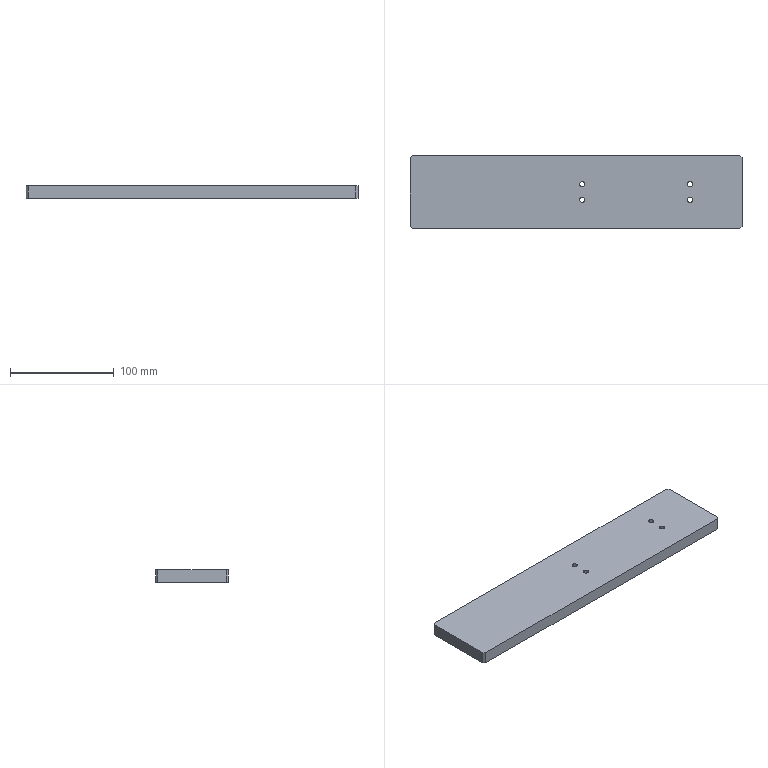Component | SolidWorks | CCDJSTransferCylinderFixingPlate01-1 | 1 solid | 58 faces | box 320 x 70 x 12 mm | volume 266860 mm3 | cylinder 28 | cone 20 | plane 10 | commonest cylinder face diameters 2.5 x10 5 x8 4.2 x6 3.3 x4 | material A6061
build123d program:
from build123d import *

# Parameters (mm, degrees)
SKETCH1_W             = 320
SKETCH1_H             = 12
BOSS_EXTRUDE1_DEPTH   = 70
CHAMFER1_SIZE         = 2
M5_TAPPED_HOLE1_D     = 4.2
M5_TAPPED_HOLE1_DEPTH = 12.4
M5_TAPPED_HOLE1_TIP   = 1.262
M4_TAPPED_HOLE1_D     = 3.3
M4_TAPPED_HOLE1_DEPTH = 10.1
M4_TAPPED_HOLE1_TIP   = 0.9914
M3_TAPPED_HOLE1_D     = 2.5
M3_TAPPED_HOLE1_DEPTH = 7.5
M3_TAPPED_HOLE1_TIP   = 0.7511
M6_TAPPED_HOLE1_D     = 5


with BuildPart() as part:
    # Sketch1 → Boss-Extrude1 (new body)
    with BuildSketch(Plane.XY):
        Rectangle(SKETCH1_W, SKETCH1_H)
    extrude(amount=BOSS_EXTRUDE1_DEPTH)

    # Chamfer1
    chamfer1_edges = [part.edges().sort_by_distance(p)[0] for p in [
        (-160, 0, 70),
        (160, 0, 70),
        (-160, 0, 0),
        (160, 0, 0),
    ]]
    chamfer(chamfer1_edges, length=CHAMFER1_SIZE)

    # M5 Tapped Hole1
    with Locations(Plane(origin=(160, 0, 0), x_dir=(0, 0, -1), z_dir=(1, 0, 0))):
        with Locations((-10, 0), (-35, 0), (-60, 0)):
            Hole(M5_TAPPED_HOLE1_D / 2, depth=M5_TAPPED_HOLE1_DEPTH)
            with Locations((0, 0, -(M5_TAPPED_HOLE1_DEPTH + M5_TAPPED_HOLE1_TIP / 2))):  # 118° drill point
                Cone(0, M5_TAPPED_HOLE1_D / 2, M5_TAPPED_HOLE1_TIP, mode=Mode.SUBTRACT)

    # M4 Tapped Hole1
    with Locations(Plane(origin=(0, 6, 0), x_dir=(1, 0, 0), z_dir=(0, 1, 0))):
        with Locations((-141, -8), (-131, -8)):
            Hole(M4_TAPPED_HOLE1_D / 2, depth=M4_TAPPED_HOLE1_DEPTH)
            with Locations((0, 0, -(M4_TAPPED_HOLE1_DEPTH + M4_TAPPED_HOLE1_TIP / 2))):  # 118° drill point
                Cone(0, M4_TAPPED_HOLE1_D / 2, M4_TAPPED_HOLE1_TIP, mode=Mode.SUBTRACT)

    # M3 Tapped Hole1
    with Locations(Plane(origin=(0, 6, 0), x_dir=(1, 0, 0), z_dir=(0, 1, 0))):
        with Locations((-139.1, -35), (-79.1, -35), (-19.1, -35), (40.9, -35), (100.9, -35)):
            Hole(M3_TAPPED_HOLE1_D / 2, depth=M3_TAPPED_HOLE1_DEPTH)
            with Locations((0, 0, -(M3_TAPPED_HOLE1_DEPTH + M3_TAPPED_HOLE1_TIP / 2))):  # 118° drill point
                Cone(0, M3_TAPPED_HOLE1_D / 2, M3_TAPPED_HOLE1_TIP, mode=Mode.SUBTRACT)

    # M6 Tapped Hole1 (through all)
    with Locations(Plane(origin=(0, -6, 0), x_dir=(-1, 0, 0), z_dir=(0, -1, 0))):
        with Locations((-110, -42.5), (-6, -42.5), (-6, -27.5), (-110, -27.5)):
            Hole(M6_TAPPED_HOLE1_D / 2)


solid = part.part

# Placed as in the assembly
solid = solid.moved(Location((-58, 391.564, -28.5), (-90, 0, 0)))